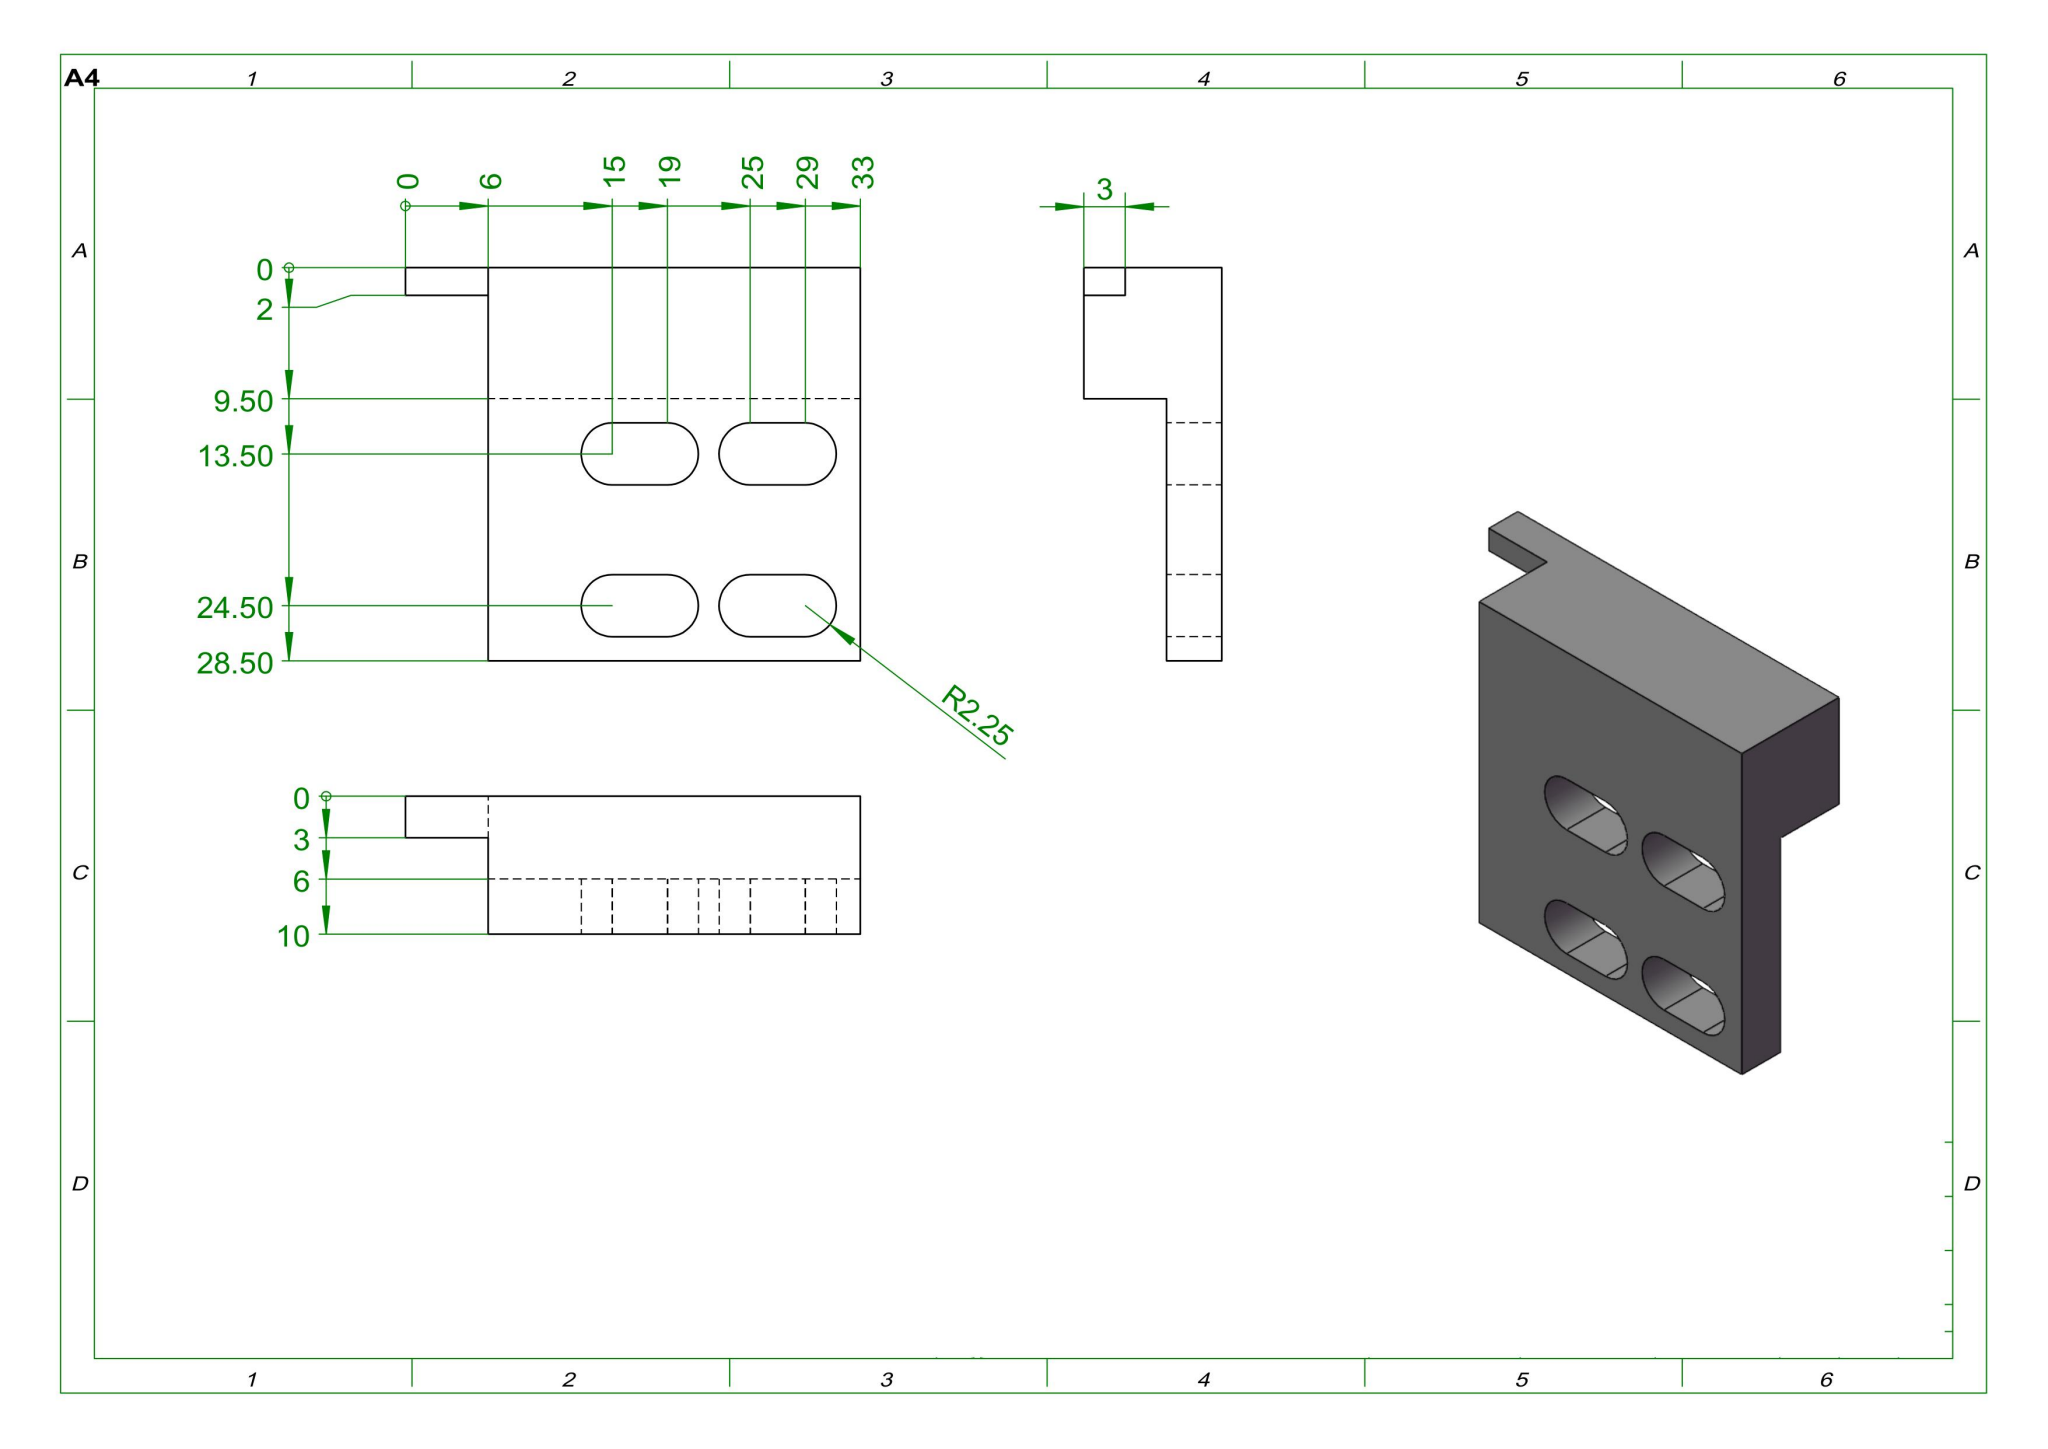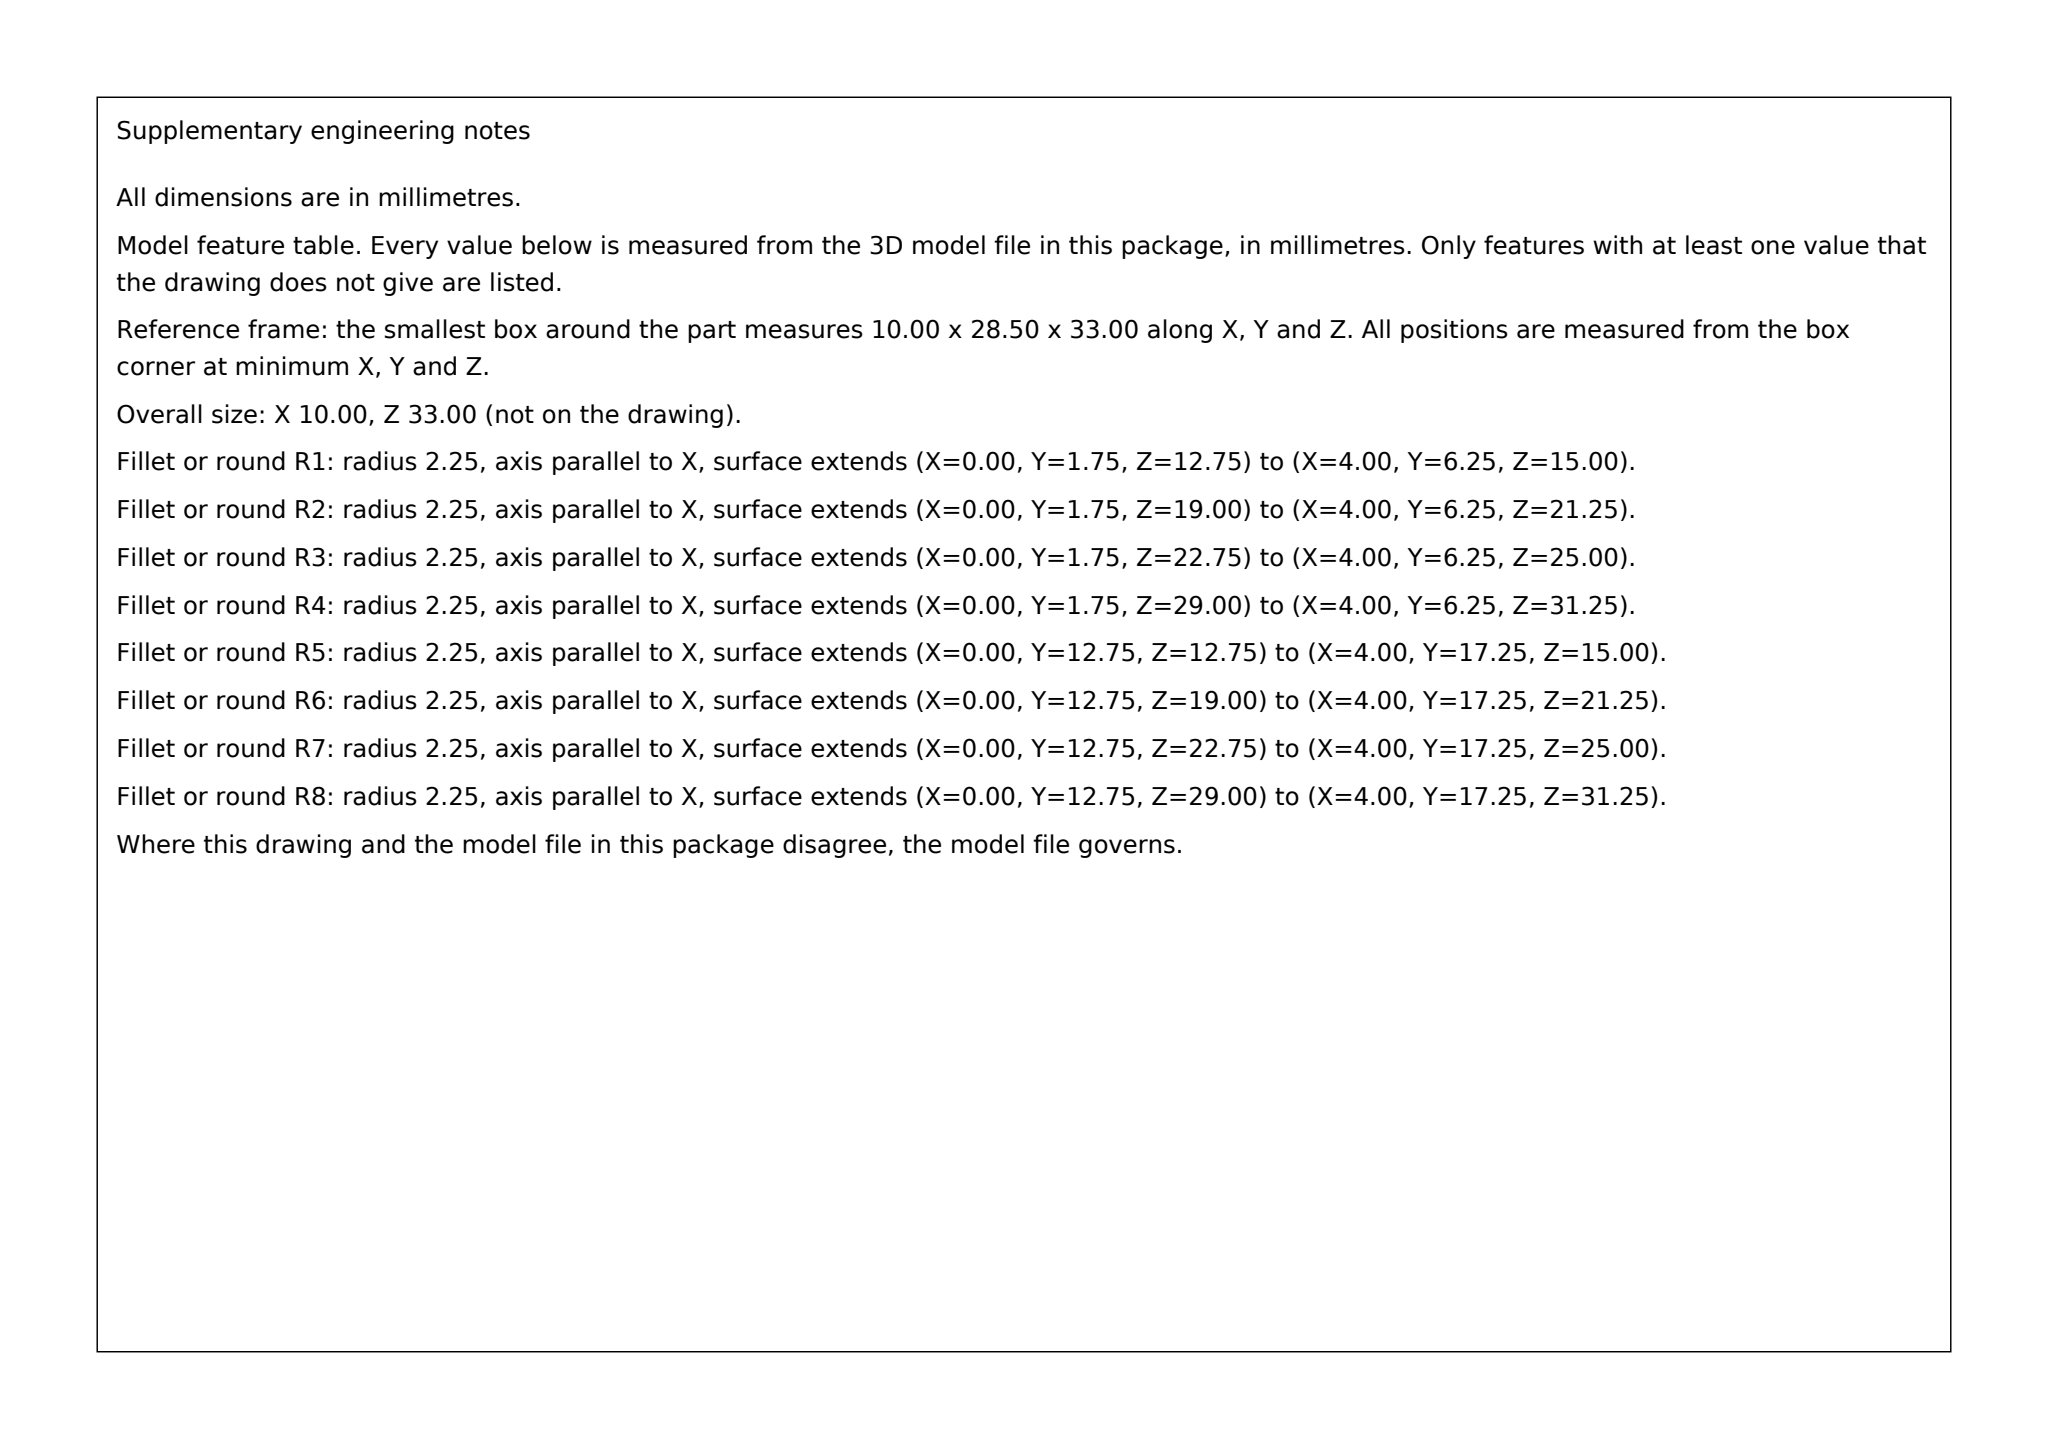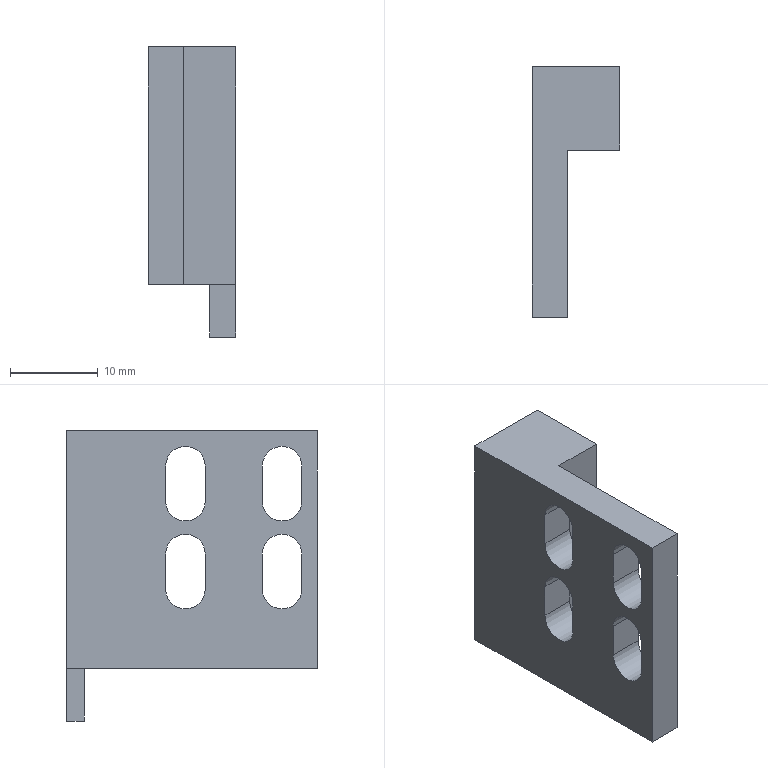Part | SolidWorks | mm | 1 solid | 27 faces | box 10 x 28.5 x 33 mm | volume 4111 mm3 | plane 19 | cylinder 8 | commonest cylinder face diameters 4.5 x8
build123d program:
from build123d import *

# Parameters (mm, degrees)
BOSS_EXTRUDE1_DEPTH = 33
CUT_EXTRUDE1_DEPTH  = 6
CUT_EXTRUDE2_DEPTH  = 10


with BuildPart() as part:
    # Sketch1 → Boss-Extrude1 (new body)
    with BuildSketch(Plane.XY):
        Polygon((0, 0), (0, 28.5), (10, 28.5), (10, 19), (4, 19), (4, 0), align=None)
    extrude(amount=BOSS_EXTRUDE1_DEPTH)

    # Sketch2 → Cut-Extrude1 (cut)
    with BuildSketch(Plane(origin=(0, 0, 0), x_dir=(-1, 0, 0), z_dir=(0, 0, -1))):
        Polygon((-7, 28.5), (-7, 26.5), (-10, 26.5), (-10, 19), (-4, 19), (-4, 0), (0, 0), (0, 28.5), align=None)
    extrude(amount=-CUT_EXTRUDE1_DEPTH, mode=Mode.SUBTRACT)

    # Sketch3 → Cut-Extrude2 (cut)
    with BuildSketch(Plane(origin=(4, 0, 0), x_dir=(0, 0, -1), z_dir=(1, 0, 0))):
        with BuildLine():
            Line((-29, 6.25), (-25, 6.25))
            ThreePointArc((-25, 6.25), (-22.75, 4), (-25, 1.75))
            Line((-25, 1.75), (-29, 1.75))
            ThreePointArc((-29, 1.75), (-31.25, 4), (-29, 6.25))
        make_face()
        with BuildLine():
            Line((-29, 12.75), (-25, 12.75))
            ThreePointArc((-25, 12.75), (-22.75, 15), (-25, 17.25))
            Line((-25, 17.25), (-29, 17.25))
            ThreePointArc((-29, 17.25), (-31.25, 15), (-29, 12.75))
        make_face()
        with BuildLine():
            Line((-19, 6.25), (-15, 6.25))
            ThreePointArc((-15, 6.25), (-12.75, 4), (-15, 1.75))
            Line((-15, 1.75), (-19, 1.75))
            ThreePointArc((-19, 1.75), (-21.25, 4), (-19, 6.25))
        make_face()
        with BuildLine():
            Line((-19, 12.75), (-15, 12.75))
            ThreePointArc((-15, 12.75), (-12.75, 15), (-15, 17.25))
            Line((-15, 17.25), (-19, 17.25))
            ThreePointArc((-19, 17.25), (-21.25, 15), (-19, 12.75))
        make_face()
    extrude(amount=-CUT_EXTRUDE2_DEPTH, mode=Mode.SUBTRACT)


solid = part.part
STEP:
#1=CARTESIAN_POINT('',(4.,-0.,6.));
#2=VERTEX_POINT('',#1);
#3=CARTESIAN_POINT('',(0.,0.,6.));
#4=VERTEX_POINT('',#3);
#5=CARTESIAN_POINT('',(4.,-0.,6.));
#6=DIRECTION('',(-1.,0.,0.));
#7=VECTOR('',#6,1000.);
#8=LINE('',#5,#7);
#9=EDGE_CURVE('',#2,#4,#8,.T.);
#10=ORIENTED_EDGE('',*,*,#9,.F.);
#11=CARTESIAN_POINT('',(4.,-0.,33.));
#12=VERTEX_POINT('',#11);
#13=CARTESIAN_POINT('',(4.,-0.,33.));
#14=DIRECTION('',(0.,0.,-1.));
#15=VECTOR('',#14,1000.);
#16=LINE('',#13,#15);
#17=EDGE_CURVE('',#12,#2,#16,.T.);
#18=ORIENTED_EDGE('',*,*,#17,.F.);
#19=CARTESIAN_POINT('',(0.,0.,33.));
#20=VERTEX_POINT('',#19);
#21=CARTESIAN_POINT('',(4.,-0.,33.));
#22=DIRECTION('',(1.,-0.,0.));
#23=VECTOR('',#22,1000.);
#24=LINE('',#21,#23);
#25=EDGE_CURVE('',#20,#12,#24,.T.);
#26=ORIENTED_EDGE('',*,*,#25,.F.);
#27=CARTESIAN_POINT('',(0.,0.,33.));
#28=DIRECTION('',(0.,0.,-1.));
#29=VECTOR('',#28,1000.);
#30=LINE('',#27,#29);
#31=EDGE_CURVE('',#20,#4,#30,.T.);
#32=ORIENTED_EDGE('',*,*,#31,.T.);
#33=EDGE_LOOP('',(#10,#18,#26,#32));
#34=FACE_OUTER_BOUND('',#33,.T.);
#35=CARTESIAN_POINT('',(4.,-0.,33.));
#36=DIRECTION('',(0.,1.,0.));
#37=DIRECTION('',(-1.,0.,0.));
#38=AXIS2_PLACEMENT_3D('',#35,#36,#37);
#39=PLANE('',#38);
#40=ADVANCED_FACE('',(#34),#39,.F.);
#41=CARTESIAN_POINT('',(4.,12.75,19.));
#42=VERTEX_POINT('',#41);
#43=CARTESIAN_POINT('',(4.,12.75,15.));
#44=VERTEX_POINT('',#43);
#45=CARTESIAN_POINT('',(4.,12.75,19.));
#46=DIRECTION('',(0.,0.,-1.));
#47=VECTOR('',#46,1000.);
#48=LINE('',#45,#47);
#49=EDGE_CURVE('',#42,#44,#48,.T.);
#50=ORIENTED_EDGE('',*,*,#49,.F.);
#51=CARTESIAN_POINT('',(4.,17.25,19.));
#52=VERTEX_POINT('',#51);
#53=CARTESIAN_POINT('',(4.,15.,19.));
#54=DIRECTION('',(1.,0.,0.));
#55=DIRECTION('',(0.,-1.,0.));
#56=AXIS2_PLACEMENT_3D('',#53,#54,#55);
#57=CIRCLE('',#56,2.25);
#58=EDGE_CURVE('',#52,#42,#57,.T.);
#59=ORIENTED_EDGE('',*,*,#58,.F.);
#60=CARTESIAN_POINT('',(4.,17.25,15.));
#61=VERTEX_POINT('',#60);
#62=CARTESIAN_POINT('',(4.,17.25,19.));
#63=DIRECTION('',(0.,0.,1.));
#64=VECTOR('',#63,1000.);
#65=LINE('',#62,#64);
#66=EDGE_CURVE('',#61,#52,#65,.T.);
#67=ORIENTED_EDGE('',*,*,#66,.F.);
#68=CARTESIAN_POINT('',(4.,15.,15.));
#69=DIRECTION('',(1.,0.,0.));
#70=DIRECTION('',(0.,-1.,0.));
#71=AXIS2_PLACEMENT_3D('',#68,#69,#70);
#72=CIRCLE('',#71,2.25);
#73=EDGE_CURVE('',#44,#61,#72,.T.);
#74=ORIENTED_EDGE('',*,*,#73,.F.);
#75=EDGE_LOOP('',(#50,#59,#67,#74));
#76=FACE_BOUND('',#75,.T.);
#77=CARTESIAN_POINT('',(4.,1.75,19.));
#78=VERTEX_POINT('',#77);
#79=CARTESIAN_POINT('',(4.,1.75,15.));
#80=VERTEX_POINT('',#79);
#81=CARTESIAN_POINT('',(4.,1.75,19.));
#82=DIRECTION('',(0.,0.,-1.));
#83=VECTOR('',#82,1000.);
#84=LINE('',#81,#83);
#85=EDGE_CURVE('',#78,#80,#84,.T.);
#86=ORIENTED_EDGE('',*,*,#85,.F.);
#87=CARTESIAN_POINT('',(4.,6.25,19.));
#88=VERTEX_POINT('',#87);
#89=CARTESIAN_POINT('',(4.,4.,19.));
#90=DIRECTION('',(1.,0.,0.));
#91=DIRECTION('',(-0.,1.,0.));
#92=AXIS2_PLACEMENT_3D('',#89,#90,#91);
#93=CIRCLE('',#92,2.25);
#94=EDGE_CURVE('',#88,#78,#93,.T.);
#95=ORIENTED_EDGE('',*,*,#94,.F.);
#96=CARTESIAN_POINT('',(4.,6.25,15.));
#97=VERTEX_POINT('',#96);
#98=CARTESIAN_POINT('',(4.,6.25,19.));
#99=DIRECTION('',(0.,0.,1.));
#100=VECTOR('',#99,1000.);
#101=LINE('',#98,#100);
#102=EDGE_CURVE('',#97,#88,#101,.T.);
#103=ORIENTED_EDGE('',*,*,#102,.F.);
#104=CARTESIAN_POINT('',(4.,4.,15.));
#105=DIRECTION('',(1.,0.,0.));
#106=DIRECTION('',(-0.,1.,0.));
#107=AXIS2_PLACEMENT_3D('',#104,#105,#106);
#108=CIRCLE('',#107,2.25);
#109=EDGE_CURVE('',#80,#97,#108,.T.);
#110=ORIENTED_EDGE('',*,*,#109,.F.);
#111=EDGE_LOOP('',(#86,#95,#103,#110));
#112=FACE_BOUND('',#111,.T.);
#113=CARTESIAN_POINT('',(4.,12.75,29.));
#114=VERTEX_POINT('',#113);
#115=CARTESIAN_POINT('',(4.,12.75,25.));
#116=VERTEX_POINT('',#115);
#117=CARTESIAN_POINT('',(4.,12.75,29.));
#118=DIRECTION('',(0.,0.,-1.));
#119=VECTOR('',#118,1000.);
#120=LINE('',#117,#119);
#121=EDGE_CURVE('',#114,#116,#120,.T.);
#122=ORIENTED_EDGE('',*,*,#121,.F.);
#123=CARTESIAN_POINT('',(4.,17.25,29.));
#124=VERTEX_POINT('',#123);
#125=CARTESIAN_POINT('',(4.,15.,29.));
#126=DIRECTION('',(1.,0.,0.));
#127=DIRECTION('',(0.,-1.,0.));
#128=AXIS2_PLACEMENT_3D('',#125,#126,#127);
#129=CIRCLE('',#128,2.25);
#130=EDGE_CURVE('',#124,#114,#129,.T.);
#131=ORIENTED_EDGE('',*,*,#130,.F.);
#132=CARTESIAN_POINT('',(4.,17.25,25.));
#133=VERTEX_POINT('',#132);
#134=CARTESIAN_POINT('',(4.,17.25,29.));
#135=DIRECTION('',(0.,0.,1.));
#136=VECTOR('',#135,1000.);
#137=LINE('',#134,#136);
#138=EDGE_CURVE('',#133,#124,#137,.T.);
#139=ORIENTED_EDGE('',*,*,#138,.F.);
#140=CARTESIAN_POINT('',(4.,15.,25.));
#141=DIRECTION('',(1.,0.,0.));
#142=DIRECTION('',(0.,-1.,0.));
#143=AXIS2_PLACEMENT_3D('',#140,#141,#142);
#144=CIRCLE('',#143,2.25);
#145=EDGE_CURVE('',#116,#133,#144,.T.);
#146=ORIENTED_EDGE('',*,*,#145,.F.);
#147=EDGE_LOOP('',(#122,#131,#139,#146));
#148=FACE_BOUND('',#147,.T.);
#149=CARTESIAN_POINT('',(4.,1.75,29.));
#150=VERTEX_POINT('',#149);
#151=CARTESIAN_POINT('',(4.,1.75,25.));
#152=VERTEX_POINT('',#151);
#153=CARTESIAN_POINT('',(4.,1.75,29.));
#154=DIRECTION('',(0.,0.,-1.));
#155=VECTOR('',#154,1000.);
#156=LINE('',#153,#155);
#157=EDGE_CURVE('',#150,#152,#156,.T.);
#158=ORIENTED_EDGE('',*,*,#157,.F.);
#159=CARTESIAN_POINT('',(4.,6.25,29.));
#160=VERTEX_POINT('',#159);
#161=CARTESIAN_POINT('',(4.,4.,29.));
#162=DIRECTION('',(1.,0.,0.));
#163=DIRECTION('',(-0.,1.,0.));
#164=AXIS2_PLACEMENT_3D('',#161,#162,#163);
#165=CIRCLE('',#164,2.25);
#166=EDGE_CURVE('',#160,#150,#165,.T.);
#167=ORIENTED_EDGE('',*,*,#166,.F.);
#168=CARTESIAN_POINT('',(4.,6.25,25.));
#169=VERTEX_POINT('',#168);
#170=CARTESIAN_POINT('',(4.,6.25,29.));
#171=DIRECTION('',(0.,0.,1.));
#172=VECTOR('',#171,1000.);
#173=LINE('',#170,#172);
#174=EDGE_CURVE('',#169,#160,#173,.T.);
#175=ORIENTED_EDGE('',*,*,#174,.F.);
#176=CARTESIAN_POINT('',(4.,4.,25.));
#177=DIRECTION('',(1.,0.,0.));
#178=DIRECTION('',(-0.,1.,0.));
#179=AXIS2_PLACEMENT_3D('',#176,#177,#178);
#180=CIRCLE('',#179,2.25);
#181=EDGE_CURVE('',#152,#169,#180,.T.);
#182=ORIENTED_EDGE('',*,*,#181,.F.);
#183=EDGE_LOOP('',(#158,#167,#175,#182));
#184=FACE_BOUND('',#183,.T.);
#185=CARTESIAN_POINT('',(4.,19.,6.));
#186=VERTEX_POINT('',#185);
#187=CARTESIAN_POINT('',(4.,19.,6.));
#188=DIRECTION('',(0.,-1.,0.));
#189=VECTOR('',#188,1000.);
#190=LINE('',#187,#189);
#191=EDGE_CURVE('',#186,#2,#190,.T.);
#192=ORIENTED_EDGE('',*,*,#191,.F.);
#193=CARTESIAN_POINT('',(4.,19.,33.));
#194=VERTEX_POINT('',#193);
#195=CARTESIAN_POINT('',(4.,19.,33.));
#196=DIRECTION('',(0.,0.,-1.));
#197=VECTOR('',#196,1000.);
#198=LINE('',#195,#197);
#199=EDGE_CURVE('',#194,#186,#198,.T.);
#200=ORIENTED_EDGE('',*,*,#199,.F.);
#201=CARTESIAN_POINT('',(4.,19.,33.));
#202=DIRECTION('',(-0.,1.,0.));
#203=VECTOR('',#202,1000.);
#204=LINE('',#201,#203);
#205=EDGE_CURVE('',#12,#194,#204,.T.);
#206=ORIENTED_EDGE('',*,*,#205,.F.);
#207=ORIENTED_EDGE('',*,*,#17,.T.);
#208=EDGE_LOOP('',(#192,#200,#206,#207));
#209=FACE_OUTER_BOUND('',#208,.T.);
#210=CARTESIAN_POINT('',(4.,19.,33.));
#211=DIRECTION('',(-1.,-0.,0.));
#212=DIRECTION('',(0.,-1.,0.));
#213=AXIS2_PLACEMENT_3D('',#210,#211,#212);
#214=PLANE('',#213);
#215=ADVANCED_FACE('',(#76,#112,#148,#184,#209),#214,.F.);
#216=CARTESIAN_POINT('',(10.,19.,6.));
#217=VERTEX_POINT('',#216);
#218=CARTESIAN_POINT('',(10.,19.,6.));
#219=DIRECTION('',(-1.,0.,0.));
#220=VECTOR('',#219,1000.);
#221=LINE('',#218,#220);
#222=EDGE_CURVE('',#217,#186,#221,.T.);
#223=ORIENTED_EDGE('',*,*,#222,.F.);
#224=CARTESIAN_POINT('',(10.,19.,33.));
#225=VERTEX_POINT('',#224);
#226=CARTESIAN_POINT('',(10.,19.,33.));
#227=DIRECTION('',(0.,0.,-1.));
#228=VECTOR('',#227,1000.);
#229=LINE('',#226,#228);
#230=EDGE_CURVE('',#225,#217,#229,.T.);
#231=ORIENTED_EDGE('',*,*,#230,.F.);
#232=CARTESIAN_POINT('',(10.,19.,33.));
#233=DIRECTION('',(1.,0.,0.));
#234=VECTOR('',#233,1000.);
#235=LINE('',#232,#234);
#236=EDGE_CURVE('',#194,#225,#235,.T.);
#237=ORIENTED_EDGE('',*,*,#236,.F.);
#238=ORIENTED_EDGE('',*,*,#199,.T.);
#239=EDGE_LOOP('',(#223,#231,#237,#238));
#240=FACE_OUTER_BOUND('',#239,.T.);
#241=CARTESIAN_POINT('',(10.,19.,33.));
#242=DIRECTION('',(0.,1.,0.));
#243=DIRECTION('',(0.,0.,1.));
#244=AXIS2_PLACEMENT_3D('',#241,#242,#243);
#245=PLANE('',#244);
#246=ADVANCED_FACE('',(#240),#245,.F.);
#247=CARTESIAN_POINT('',(0.,17.25,15.));
#248=VERTEX_POINT('',#247);
#249=CARTESIAN_POINT('',(0.,17.25,19.));
#250=VERTEX_POINT('',#249);
#251=CARTESIAN_POINT('',(0.,17.25,33.));
#252=DIRECTION('',(0.,0.,1.));
#253=VECTOR('',#252,1000.);
#254=LINE('',#251,#253);
#255=EDGE_CURVE('',#248,#250,#254,.T.);
#256=ORIENTED_EDGE('',*,*,#255,.T.);
#257=CARTESIAN_POINT('',(0.,12.75,19.));
#258=VERTEX_POINT('',#257);
#259=CARTESIAN_POINT('',(0.,15.,19.));
#260=DIRECTION('',(1.,0.,0.));
#261=DIRECTION('',(0.,0.,-1.));
#262=AXIS2_PLACEMENT_3D('',#259,#260,#261);
#263=CIRCLE('',#262,2.25);
#264=EDGE_CURVE('',#250,#258,#263,.T.);
#265=ORIENTED_EDGE('',*,*,#264,.T.);
#266=CARTESIAN_POINT('',(0.,12.75,15.));
#267=VERTEX_POINT('',#266);
#268=CARTESIAN_POINT('',(0.,12.75,33.));
#269=DIRECTION('',(0.,0.,-1.));
#270=VECTOR('',#269,1000.);
#271=LINE('',#268,#270);
#272=EDGE_CURVE('',#258,#267,#271,.T.);
#273=ORIENTED_EDGE('',*,*,#272,.T.);
#274=CARTESIAN_POINT('',(0.,15.,15.));
#275=DIRECTION('',(1.,0.,0.));
#276=DIRECTION('',(0.,0.,-1.));
#277=AXIS2_PLACEMENT_3D('',#274,#275,#276);
#278=CIRCLE('',#277,2.25);
#279=EDGE_CURVE('',#267,#248,#278,.T.);
#280=ORIENTED_EDGE('',*,*,#279,.T.);
#281=EDGE_LOOP('',(#256,#265,#273,#280));
#282=FACE_BOUND('',#281,.T.);
#283=CARTESIAN_POINT('',(0.,6.25,15.));
#284=VERTEX_POINT('',#283);
#285=CARTESIAN_POINT('',(0.,6.25,19.));
#286=VERTEX_POINT('',#285);
#287=CARTESIAN_POINT('',(0.,6.25,33.));
#288=DIRECTION('',(0.,0.,1.));
#289=VECTOR('',#288,1000.);
#290=LINE('',#287,#289);
#291=EDGE_CURVE('',#284,#286,#290,.T.);
#292=ORIENTED_EDGE('',*,*,#291,.T.);
#293=CARTESIAN_POINT('',(0.,1.75,19.));
#294=VERTEX_POINT('',#293);
#295=CARTESIAN_POINT('',(0.,4.,19.));
#296=DIRECTION('',(1.,0.,0.));
#297=DIRECTION('',(0.,0.,-1.));
#298=AXIS2_PLACEMENT_3D('',#295,#296,#297);
#299=CIRCLE('',#298,2.25);
#300=EDGE_CURVE('',#286,#294,#299,.T.);
#301=ORIENTED_EDGE('',*,*,#300,.T.);
#302=CARTESIAN_POINT('',(0.,1.75,15.));
#303=VERTEX_POINT('',#302);
#304=CARTESIAN_POINT('',(0.,1.75,33.));
#305=DIRECTION('',(0.,0.,-1.));
#306=VECTOR('',#305,1000.);
#307=LINE('',#304,#306);
#308=EDGE_CURVE('',#294,#303,#307,.T.);
#309=ORIENTED_EDGE('',*,*,#308,.T.);
#310=CARTESIAN_POINT('',(0.,4.,15.));
#311=DIRECTION('',(1.,0.,0.));
#312=DIRECTION('',(0.,0.,-1.));
#313=AXIS2_PLACEMENT_3D('',#310,#311,#312);
#314=CIRCLE('',#313,2.25);
#315=EDGE_CURVE('',#303,#284,#314,.T.);
#316=ORIENTED_EDGE('',*,*,#315,.T.);
#317=EDGE_LOOP('',(#292,#301,#309,#316));
#318=FACE_BOUND('',#317,.T.);
#319=CARTESIAN_POINT('',(0.,17.25,25.));
#320=VERTEX_POINT('',#319);
#321=CARTESIAN_POINT('',(0.,17.25,29.));
#322=VERTEX_POINT('',#321);
#323=CARTESIAN_POINT('',(0.,17.25,33.));
#324=DIRECTION('',(0.,0.,1.));
#325=VECTOR('',#324,1000.);
#326=LINE('',#323,#325);
#327=EDGE_CURVE('',#320,#322,#326,.T.);
#328=ORIENTED_EDGE('',*,*,#327,.T.);
#329=CARTESIAN_POINT('',(0.,12.75,29.));
#330=VERTEX_POINT('',#329);
#331=CARTESIAN_POINT('',(0.,15.,29.));
#332=DIRECTION('',(1.,0.,0.));
#333=DIRECTION('',(0.,0.,-1.));
#334=AXIS2_PLACEMENT_3D('',#331,#332,#333);
#335=CIRCLE('',#334,2.25);
#336=EDGE_CURVE('',#322,#330,#335,.T.);
#337=ORIENTED_EDGE('',*,*,#336,.T.);
#338=CARTESIAN_POINT('',(0.,12.75,25.));
#339=VERTEX_POINT('',#338);
#340=CARTESIAN_POINT('',(0.,12.75,33.));
#341=DIRECTION('',(0.,0.,-1.));
#342=VECTOR('',#341,1000.);
#343=LINE('',#340,#342);
#344=EDGE_CURVE('',#330,#339,#343,.T.);
#345=ORIENTED_EDGE('',*,*,#344,.T.);
#346=CARTESIAN_POINT('',(0.,15.,25.));
#347=DIRECTION('',(1.,0.,0.));
#348=DIRECTION('',(0.,0.,-1.));
#349=AXIS2_PLACEMENT_3D('',#346,#347,#348);
#350=CIRCLE('',#349,2.25);
#351=EDGE_CURVE('',#339,#320,#350,.T.);
#352=ORIENTED_EDGE('',*,*,#351,.T.);
#353=EDGE_LOOP('',(#328,#337,#345,#352));
#354=FACE_BOUND('',#353,.T.);
#355=CARTESIAN_POINT('',(0.,6.25,25.));
#356=VERTEX_POINT('',#355);
#357=CARTESIAN_POINT('',(0.,6.25,29.));
#358=VERTEX_POINT('',#357);
#359=CARTESIAN_POINT('',(0.,6.25,33.));
#360=DIRECTION('',(0.,0.,1.));
#361=VECTOR('',#360,1000.);
#362=LINE('',#359,#361);
#363=EDGE_CURVE('',#356,#358,#362,.T.);
#364=ORIENTED_EDGE('',*,*,#363,.T.);
#365=CARTESIAN_POINT('',(0.,1.75,29.));
#366=VERTEX_POINT('',#365);
#367=CARTESIAN_POINT('',(0.,4.,29.));
#368=DIRECTION('',(1.,0.,0.));
#369=DIRECTION('',(0.,0.,-1.));
#370=AXIS2_PLACEMENT_3D('',#367,#368,#369);
#371=CIRCLE('',#370,2.25);
#372=EDGE_CURVE('',#358,#366,#371,.T.);
#373=ORIENTED_EDGE('',*,*,#372,.T.);
#374=CARTESIAN_POINT('',(0.,1.75,25.));
#375=VERTEX_POINT('',#374);
#376=CARTESIAN_POINT('',(0.,1.75,33.));
#377=DIRECTION('',(0.,0.,-1.));
#378=VECTOR('',#377,1000.);
#379=LINE('',#376,#378);
#380=EDGE_CURVE('',#366,#375,#379,.T.);
#381=ORIENTED_EDGE('',*,*,#380,.T.);
#382=CARTESIAN_POINT('',(0.,4.,25.));
#383=DIRECTION('',(1.,0.,0.));
#384=DIRECTION('',(0.,0.,-1.));
#385=AXIS2_PLACEMENT_3D('',#382,#383,#384);
#386=CIRCLE('',#385,2.25);
#387=EDGE_CURVE('',#375,#356,#386,.T.);
#388=ORIENTED_EDGE('',*,*,#387,.T.);
#389=EDGE_LOOP('',(#364,#373,#381,#388));
#390=FACE_BOUND('',#389,.T.);
#391=CARTESIAN_POINT('',(0.,28.5,6.));
#392=VERTEX_POINT('',#391);
#393=CARTESIAN_POINT('',(0.,0.,6.));
#394=DIRECTION('',(0.,1.,0.));
#395=VECTOR('',#394,1000.);
#396=LINE('',#393,#395);
#397=EDGE_CURVE('',#4,#392,#396,.T.);
#398=ORIENTED_EDGE('',*,*,#397,.F.);
#399=ORIENTED_EDGE('',*,*,#31,.F.);
#400=CARTESIAN_POINT('',(0.,28.5,33.));
#401=VERTEX_POINT('',#400);
#402=CARTESIAN_POINT('',(0.,0.,33.));
#403=DIRECTION('',(0.,-1.,0.));
#404=VECTOR('',#403,1000.);
#405=LINE('',#402,#404);
#406=EDGE_CURVE('',#401,#20,#405,.T.);
#407=ORIENTED_EDGE('',*,*,#406,.F.);
#408=CARTESIAN_POINT('',(0.,28.5,33.));
#409=DIRECTION('',(0.,0.,-1.));
#410=VECTOR('',#409,1000.);
#411=LINE('',#408,#410);
#412=EDGE_CURVE('',#401,#392,#411,.T.);
#413=ORIENTED_EDGE('',*,*,#412,.T.);
#414=EDGE_LOOP('',(#398,#399,#407,#413));
#415=FACE_OUTER_BOUND('',#414,.T.);
#416=CARTESIAN_POINT('',(0.,0.,33.));
#417=DIRECTION('',(1.,0.,0.));
#418=DIRECTION('',(0.,0.,-1.));
#419=AXIS2_PLACEMENT_3D('',#416,#417,#418);
#420=PLANE('',#419);
#421=ADVANCED_FACE('',(#282,#318,#354,#390,#415),#420,.F.);
#422=CARTESIAN_POINT('',(10.,26.5,6.));
#423=VERTEX_POINT('',#422);
#424=CARTESIAN_POINT('',(10.,26.5,6.));
#425=DIRECTION('',(0.,-1.,0.));
#426=VECTOR('',#425,1000.);
#427=LINE('',#424,#426);
#428=EDGE_CURVE('',#423,#217,#427,.T.);
#429=ORIENTED_EDGE('',*,*,#428,.F.);
#430=CARTESIAN_POINT('',(10.,26.5,0.));
#431=VERTEX_POINT('',#430);
#432=CARTESIAN_POINT('',(10.,26.5,6.));
#433=DIRECTION('',(0.,0.,-1.));
#434=VECTOR('',#433,1000.);
#435=LINE('',#432,#434);
#436=EDGE_CURVE('',#423,#431,#435,.T.);
#437=ORIENTED_EDGE('',*,*,#436,.T.);
#438=CARTESIAN_POINT('',(10.,28.5,0.));
#439=VERTEX_POINT('',#438);
#440=CARTESIAN_POINT('',(10.,28.5,0.));
#441=DIRECTION('',(-0.,1.,0.));
#442=VECTOR('',#441,1000.);
#443=LINE('',#440,#442);
#444=EDGE_CURVE('',#431,#439,#443,.T.);
#445=ORIENTED_EDGE('',*,*,#444,.T.);
#446=CARTESIAN_POINT('',(10.,28.5,33.));
#447=VERTEX_POINT('',#446);
#448=CARTESIAN_POINT('',(10.,28.5,33.));
#449=DIRECTION('',(0.,0.,-1.));
#450=VECTOR('',#449,1000.);
#451=LINE('',#448,#450);
#452=EDGE_CURVE('',#447,#439,#451,.T.);
#453=ORIENTED_EDGE('',*,*,#452,.F.);
#454=CARTESIAN_POINT('',(10.,28.5,33.));
#455=DIRECTION('',(-0.,1.,0.));
#456=VECTOR('',#455,1000.);
#457=LINE('',#454,#456);
#458=EDGE_CURVE('',#225,#447,#457,.T.);
#459=ORIENTED_EDGE('',*,*,#458,.F.);
#460=ORIENTED_EDGE('',*,*,#230,.T.);
#461=EDGE_LOOP('',(#429,#437,#445,#453,#459,#460));
#462=FACE_OUTER_BOUND('',#461,.T.);
#463=CARTESIAN_POINT('',(10.,28.5,33.));
#464=DIRECTION('',(-1.,-0.,0.));
#465=DIRECTION('',(0.,-1.,0.));
#466=AXIS2_PLACEMENT_3D('',#463,#464,#465);
#467=PLANE('',#466);
#468=ADVANCED_FACE('',(#462),#467,.F.);
#469=CARTESIAN_POINT('',(7.,28.5,0.));
#470=VERTEX_POINT('',#469);
#471=CARTESIAN_POINT('',(0.,28.5,0.));
#472=DIRECTION('',(-1.,0.,0.));
#473=VECTOR('',#472,1000.);
#474=LINE('',#471,#473);
#475=EDGE_CURVE('',#439,#470,#474,.T.);
#476=ORIENTED_EDGE('',*,*,#475,.T.);
#477=CARTESIAN_POINT('',(7.,28.5,6.));
#478=VERTEX_POINT('',#477);
#479=CARTESIAN_POINT('',(7.,28.5,6.));
#480=DIRECTION('',(0.,0.,-1.));
#481=VECTOR('',#480,1000.);
#482=LINE('',#479,#481);
#483=EDGE_CURVE('',#478,#470,#482,.T.);
#484=ORIENTED_EDGE('',*,*,#483,.F.);
#485=CARTESIAN_POINT('',(0.,28.5,6.));
#486=DIRECTION('',(1.,0.,0.));
#487=VECTOR('',#486,1000.);
#488=LINE('',#485,#487);
#489=EDGE_CURVE('',#392,#478,#488,.T.);
#490=ORIENTED_EDGE('',*,*,#489,.F.);
#491=ORIENTED_EDGE('',*,*,#412,.F.);
#492=CARTESIAN_POINT('',(0.,28.5,33.));
#493=DIRECTION('',(-1.,0.,0.));
#494=VECTOR('',#493,1000.);
#495=LINE('',#492,#494);
#496=EDGE_CURVE('',#447,#401,#495,.T.);
#497=ORIENTED_EDGE('',*,*,#496,.F.);
#498=ORIENTED_EDGE('',*,*,#452,.T.);
#499=EDGE_LOOP('',(#476,#484,#490,#491,#497,#498));
#500=FACE_OUTER_BOUND('',#499,.T.);
#501=CARTESIAN_POINT('',(0.,28.5,33.));
#502=DIRECTION('',(0.,-1.,0.));
#503=DIRECTION('',(0.,0.,-1.));
#504=AXIS2_PLACEMENT_3D('',#501,#502,#503);
#505=PLANE('',#504);
#506=ADVANCED_FACE('',(#500),#505,.F.);
#507=ORIENTED_EDGE('',*,*,#25,.T.);
#508=ORIENTED_EDGE('',*,*,#205,.T.);
#509=ORIENTED_EDGE('',*,*,#236,.T.);
#510=ORIENTED_EDGE('',*,*,#458,.T.);
#511=ORIENTED_EDGE('',*,*,#496,.T.);
#512=ORIENTED_EDGE('',*,*,#406,.T.);
#513=EDGE_LOOP('',(#507,#508,#509,#510,#511,#512));
#514=FACE_OUTER_BOUND('',#513,.T.);
#515=CARTESIAN_POINT('',(0.,0.,33.));
#516=DIRECTION('',(0.,0.,-1.));
#517=DIRECTION('',(-1.,0.,0.));
#518=AXIS2_PLACEMENT_3D('',#515,#516,#517);
#519=PLANE('',#518);
#520=ADVANCED_FACE('',(#514),#519,.F.);
#521=CARTESIAN_POINT('',(7.,26.5,0.));
#522=VERTEX_POINT('',#521);
#523=CARTESIAN_POINT('',(7.,26.5,0.));
#524=DIRECTION('',(1.,0.,0.));
#525=VECTOR('',#524,1000.);
#526=LINE('',#523,#525);
#527=EDGE_CURVE('',#522,#431,#526,.T.);
#528=ORIENTED_EDGE('',*,*,#527,.F.);
#529=CARTESIAN_POINT('',(7.,28.5,0.));
#530=DIRECTION('',(-0.,-1.,0.));
#531=VECTOR('',#530,1000.);
#532=LINE('',#529,#531);
#533=EDGE_CURVE('',#470,#522,#532,.T.);
#534=ORIENTED_EDGE('',*,*,#533,.F.);
#535=ORIENTED_EDGE('',*,*,#475,.F.);
#536=ORIENTED_EDGE('',*,*,#444,.F.);
#537=EDGE_LOOP('',(#528,#534,#535,#536));
#538=FACE_OUTER_BOUND('',#537,.T.);
#539=CARTESIAN_POINT('',(0.,0.,0.));
#540=DIRECTION('',(0.,0.,-1.));
#541=DIRECTION('',(-1.,0.,0.));
#542=AXIS2_PLACEMENT_3D('',#539,#540,#541);
#543=PLANE('',#542);
#544=ADVANCED_FACE('',(#538),#543,.T.);
#545=ORIENTED_EDGE('',*,*,#527,.T.);
#546=ORIENTED_EDGE('',*,*,#436,.F.);
#547=CARTESIAN_POINT('',(7.,26.5,6.));
#548=VERTEX_POINT('',#547);
#549=CARTESIAN_POINT('',(7.,26.5,6.));
#550=DIRECTION('',(1.,0.,0.));
#551=VECTOR('',#550,1000.);
#552=LINE('',#549,#551);
#553=EDGE_CURVE('',#548,#423,#552,.T.);
#554=ORIENTED_EDGE('',*,*,#553,.F.);
#555=CARTESIAN_POINT('',(7.,26.5,6.));
#556=DIRECTION('',(0.,0.,-1.));
#557=VECTOR('',#556,1000.);
#558=LINE('',#555,#557);
#559=EDGE_CURVE('',#548,#522,#558,.T.);
#560=ORIENTED_EDGE('',*,*,#559,.T.);
#561=EDGE_LOOP('',(#545,#546,#554,#560));
#562=FACE_OUTER_BOUND('',#561,.T.);
#563=CARTESIAN_POINT('',(7.,26.5,6.));
#564=DIRECTION('',(0.,1.,0.));
#565=DIRECTION('',(0.,0.,1.));
#566=AXIS2_PLACEMENT_3D('',#563,#564,#565);
#567=PLANE('',#566);
#568=ADVANCED_FACE('',(#562),#567,.F.);
#569=ORIENTED_EDGE('',*,*,#533,.T.);
#570=ORIENTED_EDGE('',*,*,#559,.F.);
#571=CARTESIAN_POINT('',(7.,28.5,6.));
#572=DIRECTION('',(-0.,-1.,0.));
#573=VECTOR('',#572,1000.);
#574=LINE('',#571,#573);
#575=EDGE_CURVE('',#478,#548,#574,.T.);
#576=ORIENTED_EDGE('',*,*,#575,.F.);
#577=ORIENTED_EDGE('',*,*,#483,.T.);
#578=EDGE_LOOP('',(#569,#570,#576,#577));
#579=FACE_OUTER_BOUND('',#578,.T.);
#580=CARTESIAN_POINT('',(7.,28.5,6.));
#581=DIRECTION('',(1.,-0.,0.));
#582=DIRECTION('',(0.,1.,0.));
#583=AXIS2_PLACEMENT_3D('',#580,#581,#582);
#584=PLANE('',#583);
#585=ADVANCED_FACE('',(#579),#584,.F.);
#586=ORIENTED_EDGE('',*,*,#489,.T.);
#587=ORIENTED_EDGE('',*,*,#575,.T.);
#588=ORIENTED_EDGE('',*,*,#553,.T.);
#589=ORIENTED_EDGE('',*,*,#428,.T.);
#590=ORIENTED_EDGE('',*,*,#222,.T.);
#591=ORIENTED_EDGE('',*,*,#191,.T.);
#592=ORIENTED_EDGE('',*,*,#9,.T.);
#593=ORIENTED_EDGE('',*,*,#397,.T.);
#594=EDGE_LOOP('',(#586,#587,#588,#589,#590,#591,#592,#593));
#595=FACE_OUTER_BOUND('',#594,.T.);
#596=CARTESIAN_POINT('',(0.,0.,6.));
#597=DIRECTION('',(0.,0.,-1.));
#598=DIRECTION('',(-1.,0.,0.));
#599=AXIS2_PLACEMENT_3D('',#596,#597,#598);
#600=PLANE('',#599);
#601=ADVANCED_FACE('',(#595),#600,.T.);
#602=CARTESIAN_POINT('',(-6.,6.25,29.));
#603=DIRECTION('',(1.,0.,0.));
#604=VECTOR('',#603,1000.);
#605=LINE('',#602,#604);
#606=EDGE_CURVE('',#358,#160,#605,.T.);
#607=ORIENTED_EDGE('',*,*,#606,.T.);
#608=ORIENTED_EDGE('',*,*,#166,.T.);
#609=CARTESIAN_POINT('',(-6.,1.75,29.));
#610=DIRECTION('',(1.,0.,0.));
#611=VECTOR('',#610,1000.);
#612=LINE('',#609,#611);
#613=EDGE_CURVE('',#366,#150,#612,.T.);
#614=ORIENTED_EDGE('',*,*,#613,.F.);
#615=ORIENTED_EDGE('',*,*,#372,.F.);
#616=EDGE_LOOP('',(#607,#608,#614,#615));
#617=FACE_OUTER_BOUND('',#616,.T.);
#618=CARTESIAN_POINT('',(-6.,4.,29.));
#619=DIRECTION('',(1.,0.,0.));
#620=DIRECTION('',(-0.,1.,0.));
#621=AXIS2_PLACEMENT_3D('',#618,#619,#620);
#622=CYLINDRICAL_SURFACE('',#621,2.25);
#623=ADVANCED_FACE('',(#617),#622,.F.);
#624=CARTESIAN_POINT('',(-6.,6.25,25.));
#625=DIRECTION('',(1.,0.,0.));
#626=VECTOR('',#625,1000.);
#627=LINE('',#624,#626);
#628=EDGE_CURVE('',#356,#169,#627,.T.);
#629=ORIENTED_EDGE('',*,*,#628,.T.);
#630=ORIENTED_EDGE('',*,*,#174,.T.);
#631=ORIENTED_EDGE('',*,*,#606,.F.);
#632=ORIENTED_EDGE('',*,*,#363,.F.);
#633=EDGE_LOOP('',(#629,#630,#631,#632));
#634=FACE_OUTER_BOUND('',#633,.T.);
#635=CARTESIAN_POINT('',(-6.,6.25,29.));
#636=DIRECTION('',(-0.,1.,0.));
#637=DIRECTION('',(-1.,-0.,0.));
#638=AXIS2_PLACEMENT_3D('',#635,#636,#637);
#639=PLANE('',#638);
#640=ADVANCED_FACE('',(#634),#639,.F.);
#641=CARTESIAN_POINT('',(-6.,1.75,25.));
#642=DIRECTION('',(1.,0.,0.));
#643=VECTOR('',#642,1000.);
#644=LINE('',#641,#643);
#645=EDGE_CURVE('',#375,#152,#644,.T.);
#646=ORIENTED_EDGE('',*,*,#645,.T.);
#647=ORIENTED_EDGE('',*,*,#181,.T.);
#648=ORIENTED_EDGE('',*,*,#628,.F.);
#649=ORIENTED_EDGE('',*,*,#387,.F.);
#650=EDGE_LOOP('',(#646,#647,#648,#649));
#651=FACE_OUTER_BOUND('',#650,.T.);
#652=CARTESIAN_POINT('',(-6.,4.,25.));
#653=DIRECTION('',(1.,0.,0.));
#654=DIRECTION('',(-0.,1.,0.));
#655=AXIS2_PLACEMENT_3D('',#652,#653,#654);
#656=CYLINDRICAL_SURFACE('',#655,2.25);
#657=ADVANCED_FACE('',(#651),#656,.F.);
#658=ORIENTED_EDGE('',*,*,#613,.T.);
#659=ORIENTED_EDGE('',*,*,#157,.T.);
#660=ORIENTED_EDGE('',*,*,#645,.F.);
#661=ORIENTED_EDGE('',*,*,#380,.F.);
#662=EDGE_LOOP('',(#658,#659,#660,#661));
#663=FACE_OUTER_BOUND('',#662,.T.);
#664=CARTESIAN_POINT('',(-6.,1.75,29.));
#665=DIRECTION('',(0.,-1.,0.));
#666=DIRECTION('',(1.,0.,0.));
#667=AXIS2_PLACEMENT_3D('',#664,#665,#666);
#668=PLANE('',#667);
#669=ADVANCED_FACE('',(#663),#668,.F.);
#670=CARTESIAN_POINT('',(-6.,17.25,29.));
#671=DIRECTION('',(1.,0.,0.));
#672=VECTOR('',#671,1000.);
#673=LINE('',#670,#672);
#674=EDGE_CURVE('',#322,#124,#673,.T.);
#675=ORIENTED_EDGE('',*,*,#674,.T.);
#676=ORIENTED_EDGE('',*,*,#130,.T.);
#677=CARTESIAN_POINT('',(-6.,12.75,29.));
#678=DIRECTION('',(1.,0.,0.));
#679=VECTOR('',#678,1000.);
#680=LINE('',#677,#679);
#681=EDGE_CURVE('',#330,#114,#680,.T.);
#682=ORIENTED_EDGE('',*,*,#681,.F.);
#683=ORIENTED_EDGE('',*,*,#336,.F.);
#684=EDGE_LOOP('',(#675,#676,#682,#683));
#685=FACE_OUTER_BOUND('',#684,.T.);
#686=CARTESIAN_POINT('',(-6.,15.,29.));
#687=DIRECTION('',(1.,0.,0.));
#688=DIRECTION('',(-0.,1.,0.));
#689=AXIS2_PLACEMENT_3D('',#686,#687,#688);
#690=CYLINDRICAL_SURFACE('',#689,2.25);
#691=ADVANCED_FACE('',(#685),#690,.F.);
#692=CARTESIAN_POINT('',(-6.,17.25,25.));
#693=DIRECTION('',(1.,0.,0.));
#694=VECTOR('',#693,1000.);
#695=LINE('',#692,#694);
#696=EDGE_CURVE('',#320,#133,#695,.T.);
#697=ORIENTED_EDGE('',*,*,#696,.T.);
#698=ORIENTED_EDGE('',*,*,#138,.T.);
#699=ORIENTED_EDGE('',*,*,#674,.F.);
#700=ORIENTED_EDGE('',*,*,#327,.F.);
#701=EDGE_LOOP('',(#697,#698,#699,#700));
#702=FACE_OUTER_BOUND('',#701,.T.);
#703=CARTESIAN_POINT('',(-6.,17.25,29.));
#704=DIRECTION('',(-0.,1.,0.));
#705=DIRECTION('',(-1.,-0.,0.));
#706=AXIS2_PLACEMENT_3D('',#703,#704,#705);
#707=PLANE('',#706);
#708=ADVANCED_FACE('',(#702),#707,.F.);
#709=CARTESIAN_POINT('',(-6.,12.75,25.));
#710=DIRECTION('',(1.,0.,0.));
#711=VECTOR('',#710,1000.);
#712=LINE('',#709,#711);
#713=EDGE_CURVE('',#339,#116,#712,.T.);
#714=ORIENTED_EDGE('',*,*,#713,.T.);
#715=ORIENTED_EDGE('',*,*,#145,.T.);
#716=ORIENTED_EDGE('',*,*,#696,.F.);
#717=ORIENTED_EDGE('',*,*,#351,.F.);
#718=EDGE_LOOP('',(#714,#715,#716,#717));
#719=FACE_OUTER_BOUND('',#718,.T.);
#720=CARTESIAN_POINT('',(-6.,15.,25.));
#721=DIRECTION('',(1.,0.,0.));
#722=DIRECTION('',(-0.,1.,0.));
#723=AXIS2_PLACEMENT_3D('',#720,#721,#722);
#724=CYLINDRICAL_SURFACE('',#723,2.25);
#725=ADVANCED_FACE('',(#719),#724,.F.);
#726=ORIENTED_EDGE('',*,*,#681,.T.);
#727=ORIENTED_EDGE('',*,*,#121,.T.);
#728=ORIENTED_EDGE('',*,*,#713,.F.);
#729=ORIENTED_EDGE('',*,*,#344,.F.);
#730=EDGE_LOOP('',(#726,#727,#728,#729));
#731=FACE_OUTER_BOUND('',#730,.T.);
#732=CARTESIAN_POINT('',(-6.,12.75,29.));
#733=DIRECTION('',(0.,-1.,0.));
#734=DIRECTION('',(1.,0.,0.));
#735=AXIS2_PLACEMENT_3D('',#732,#733,#734);
#736=PLANE('',#735);
#737=ADVANCED_FACE('',(#731),#736,.F.);
#738=CARTESIAN_POINT('',(-6.,6.25,19.));
#739=DIRECTION('',(1.,0.,0.));
#740=VECTOR('',#739,1000.);
#741=LINE('',#738,#740);
#742=EDGE_CURVE('',#286,#88,#741,.T.);
#743=ORIENTED_EDGE('',*,*,#742,.T.);
#744=ORIENTED_EDGE('',*,*,#94,.T.);
#745=CARTESIAN_POINT('',(-6.,1.75,19.));
#746=DIRECTION('',(1.,0.,0.));
#747=VECTOR('',#746,1000.);
#748=LINE('',#745,#747);
#749=EDGE_CURVE('',#294,#78,#748,.T.);
#750=ORIENTED_EDGE('',*,*,#749,.F.);
#751=ORIENTED_EDGE('',*,*,#300,.F.);
#752=EDGE_LOOP('',(#743,#744,#750,#751));
#753=FACE_OUTER_BOUND('',#752,.T.);
#754=CARTESIAN_POINT('',(-6.,4.,19.));
#755=DIRECTION('',(1.,0.,0.));
#756=DIRECTION('',(-0.,1.,0.));
#757=AXIS2_PLACEMENT_3D('',#754,#755,#756);
#758=CYLINDRICAL_SURFACE('',#757,2.25);
#759=ADVANCED_FACE('',(#753),#758,.F.);
#760=CARTESIAN_POINT('',(-6.,6.25,15.));
#761=DIRECTION('',(1.,0.,0.));
#762=VECTOR('',#761,1000.);
#763=LINE('',#760,#762);
#764=EDGE_CURVE('',#284,#97,#763,.T.);
#765=ORIENTED_EDGE('',*,*,#764,.T.);
#766=ORIENTED_EDGE('',*,*,#102,.T.);
#767=ORIENTED_EDGE('',*,*,#742,.F.);
#768=ORIENTED_EDGE('',*,*,#291,.F.);
#769=EDGE_LOOP('',(#765,#766,#767,#768));
#770=FACE_OUTER_BOUND('',#769,.T.);
#771=CARTESIAN_POINT('',(-6.,6.25,19.));
#772=DIRECTION('',(-0.,1.,0.));
#773=DIRECTION('',(-1.,-0.,0.));
#774=AXIS2_PLACEMENT_3D('',#771,#772,#773);
#775=PLANE('',#774);
#776=ADVANCED_FACE('',(#770),#775,.F.);
#777=CARTESIAN_POINT('',(-6.,1.75,15.));
#778=DIRECTION('',(1.,0.,0.));
#779=VECTOR('',#778,1000.);
#780=LINE('',#777,#779);
#781=EDGE_CURVE('',#303,#80,#780,.T.);
#782=ORIENTED_EDGE('',*,*,#781,.T.);
#783=ORIENTED_EDGE('',*,*,#109,.T.);
#784=ORIENTED_EDGE('',*,*,#764,.F.);
#785=ORIENTED_EDGE('',*,*,#315,.F.);
#786=EDGE_LOOP('',(#782,#783,#784,#785));
#787=FACE_OUTER_BOUND('',#786,.T.);
#788=CARTESIAN_POINT('',(-6.,4.,15.));
#789=DIRECTION('',(1.,0.,0.));
#790=DIRECTION('',(-0.,1.,0.));
#791=AXIS2_PLACEMENT_3D('',#788,#789,#790);
#792=CYLINDRICAL_SURFACE('',#791,2.25);
#793=ADVANCED_FACE('',(#787),#792,.F.);
#794=ORIENTED_EDGE('',*,*,#749,.T.);
#795=ORIENTED_EDGE('',*,*,#85,.T.);
#796=ORIENTED_EDGE('',*,*,#781,.F.);
#797=ORIENTED_EDGE('',*,*,#308,.F.);
#798=EDGE_LOOP('',(#794,#795,#796,#797));
#799=FACE_OUTER_BOUND('',#798,.T.);
#800=CARTESIAN_POINT('',(-6.,1.75,19.));
#801=DIRECTION('',(0.,-1.,0.));
#802=DIRECTION('',(1.,0.,0.));
#803=AXIS2_PLACEMENT_3D('',#800,#801,#802);
#804=PLANE('',#803);
#805=ADVANCED_FACE('',(#799),#804,.F.);
#806=CARTESIAN_POINT('',(-6.,17.25,19.));
#807=DIRECTION('',(1.,0.,0.));
#808=VECTOR('',#807,1000.);
#809=LINE('',#806,#808);
#810=EDGE_CURVE('',#250,#52,#809,.T.);
#811=ORIENTED_EDGE('',*,*,#810,.T.);
#812=ORIENTED_EDGE('',*,*,#58,.T.);
#813=CARTESIAN_POINT('',(-6.,12.75,19.));
#814=DIRECTION('',(1.,0.,0.));
#815=VECTOR('',#814,1000.);
#816=LINE('',#813,#815);
#817=EDGE_CURVE('',#258,#42,#816,.T.);
#818=ORIENTED_EDGE('',*,*,#817,.F.);
#819=ORIENTED_EDGE('',*,*,#264,.F.);
#820=EDGE_LOOP('',(#811,#812,#818,#819));
#821=FACE_OUTER_BOUND('',#820,.T.);
#822=CARTESIAN_POINT('',(-6.,15.,19.));
#823=DIRECTION('',(1.,0.,0.));
#824=DIRECTION('',(-0.,1.,0.));
#825=AXIS2_PLACEMENT_3D('',#822,#823,#824);
#826=CYLINDRICAL_SURFACE('',#825,2.25);
#827=ADVANCED_FACE('',(#821),#826,.F.);
#828=CARTESIAN_POINT('',(-6.,17.25,15.));
#829=DIRECTION('',(1.,0.,0.));
#830=VECTOR('',#829,1000.);
#831=LINE('',#828,#830);
#832=EDGE_CURVE('',#248,#61,#831,.T.);
#833=ORIENTED_EDGE('',*,*,#832,.T.);
#834=ORIENTED_EDGE('',*,*,#66,.T.);
#835=ORIENTED_EDGE('',*,*,#810,.F.);
#836=ORIENTED_EDGE('',*,*,#255,.F.);
#837=EDGE_LOOP('',(#833,#834,#835,#836));
#838=FACE_OUTER_BOUND('',#837,.T.);
#839=CARTESIAN_POINT('',(-6.,17.25,19.));
#840=DIRECTION('',(-0.,1.,0.));
#841=DIRECTION('',(-1.,-0.,0.));
#842=AXIS2_PLACEMENT_3D('',#839,#840,#841);
#843=PLANE('',#842);
#844=ADVANCED_FACE('',(#838),#843,.F.);
#845=CARTESIAN_POINT('',(-6.,12.75,15.));
#846=DIRECTION('',(1.,0.,0.));
#847=VECTOR('',#846,1000.);
#848=LINE('',#845,#847);
#849=EDGE_CURVE('',#267,#44,#848,.T.);
#850=ORIENTED_EDGE('',*,*,#849,.T.);
#851=ORIENTED_EDGE('',*,*,#73,.T.);
#852=ORIENTED_EDGE('',*,*,#832,.F.);
#853=ORIENTED_EDGE('',*,*,#279,.F.);
#854=EDGE_LOOP('',(#850,#851,#852,#853));
#855=FACE_OUTER_BOUND('',#854,.T.);
#856=CARTESIAN_POINT('',(-6.,15.,15.));
#857=DIRECTION('',(1.,0.,0.));
#858=DIRECTION('',(-0.,1.,0.));
#859=AXIS2_PLACEMENT_3D('',#856,#857,#858);
#860=CYLINDRICAL_SURFACE('',#859,2.25);
#861=ADVANCED_FACE('',(#855),#860,.F.);
#862=ORIENTED_EDGE('',*,*,#817,.T.);
#863=ORIENTED_EDGE('',*,*,#49,.T.);
#864=ORIENTED_EDGE('',*,*,#849,.F.);
#865=ORIENTED_EDGE('',*,*,#272,.F.);
#866=EDGE_LOOP('',(#862,#863,#864,#865));
#867=FACE_OUTER_BOUND('',#866,.T.);
#868=CARTESIAN_POINT('',(-6.,12.75,19.));
#869=DIRECTION('',(0.,-1.,0.));
#870=DIRECTION('',(1.,0.,0.));
#871=AXIS2_PLACEMENT_3D('',#868,#869,#870);
#872=PLANE('',#871);
#873=ADVANCED_FACE('',(#867),#872,.F.);
#874=CLOSED_SHELL('',(#40,#215,#246,#421,#468,#506,#520,#544,#568,#585,#601,#623,#640,#657,#669,#691,#708,#725,#737,#759,#776,#793,#805,#827,#844,#861,#873));
#875=MANIFOLD_SOLID_BREP('',#874);
#876=CARTESIAN_POINT('',(0.,0.,0.));
#877=DIRECTION('',(0.,0.,1.));
#878=DIRECTION('',(1.,0.,0.));
#879=AXIS2_PLACEMENT_3D('',#876,#877,#878);
#880=(LENGTH_UNIT()NAMED_UNIT(*)SI_UNIT(.MILLI.,.METRE.));
#881=UNCERTAINTY_MEASURE_WITH_UNIT(LENGTH_MEASURE(0.00001),#880,'','');
#882=(NAMED_UNIT(*)PLANE_ANGLE_UNIT()SI_UNIT($,.RADIAN.));
#883=(NAMED_UNIT(*)SI_UNIT($,.STERADIAN.)SOLID_ANGLE_UNIT());
#884=(GEOMETRIC_REPRESENTATION_CONTEXT(3)GLOBAL_UNCERTAINTY_ASSIGNED_CONTEXT((#881))GLOBAL_UNIT_ASSIGNED_CONTEXT((#880,#882,#883))REPRESENTATION_CONTEXT('',''));
#885=ADVANCED_BREP_SHAPE_REPRESENTATION('',(#875,#879),#884);